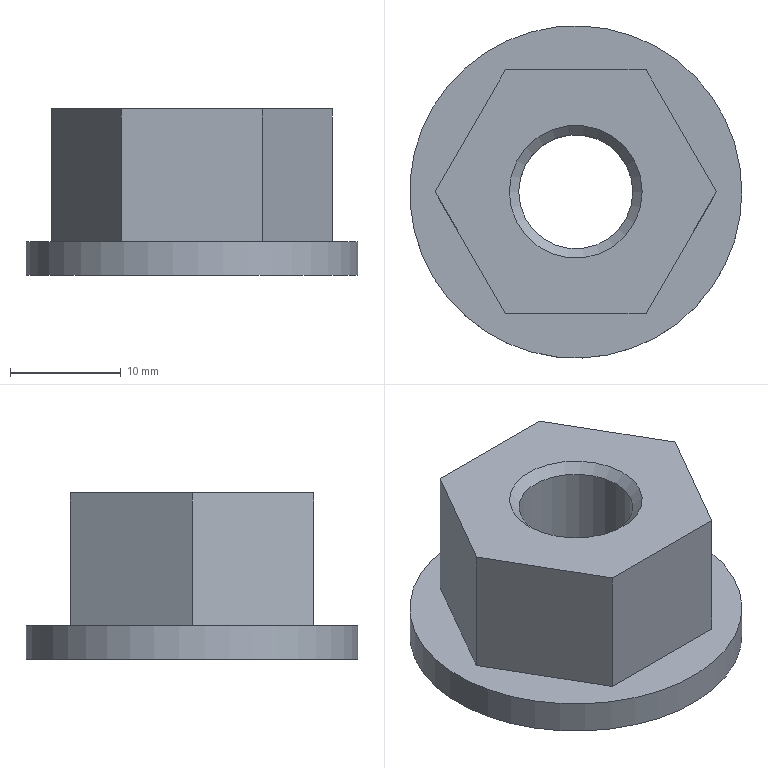CAM job | NX | mm | 3-axis | 1 set-up | 1 operations | part box 30 x 30 x 15
set-up 1
1. Cavity Milling | Mill Mill5 MILLMILL_D10 | CAVITY_MILL | path 8458.903 mm | 15.138 min